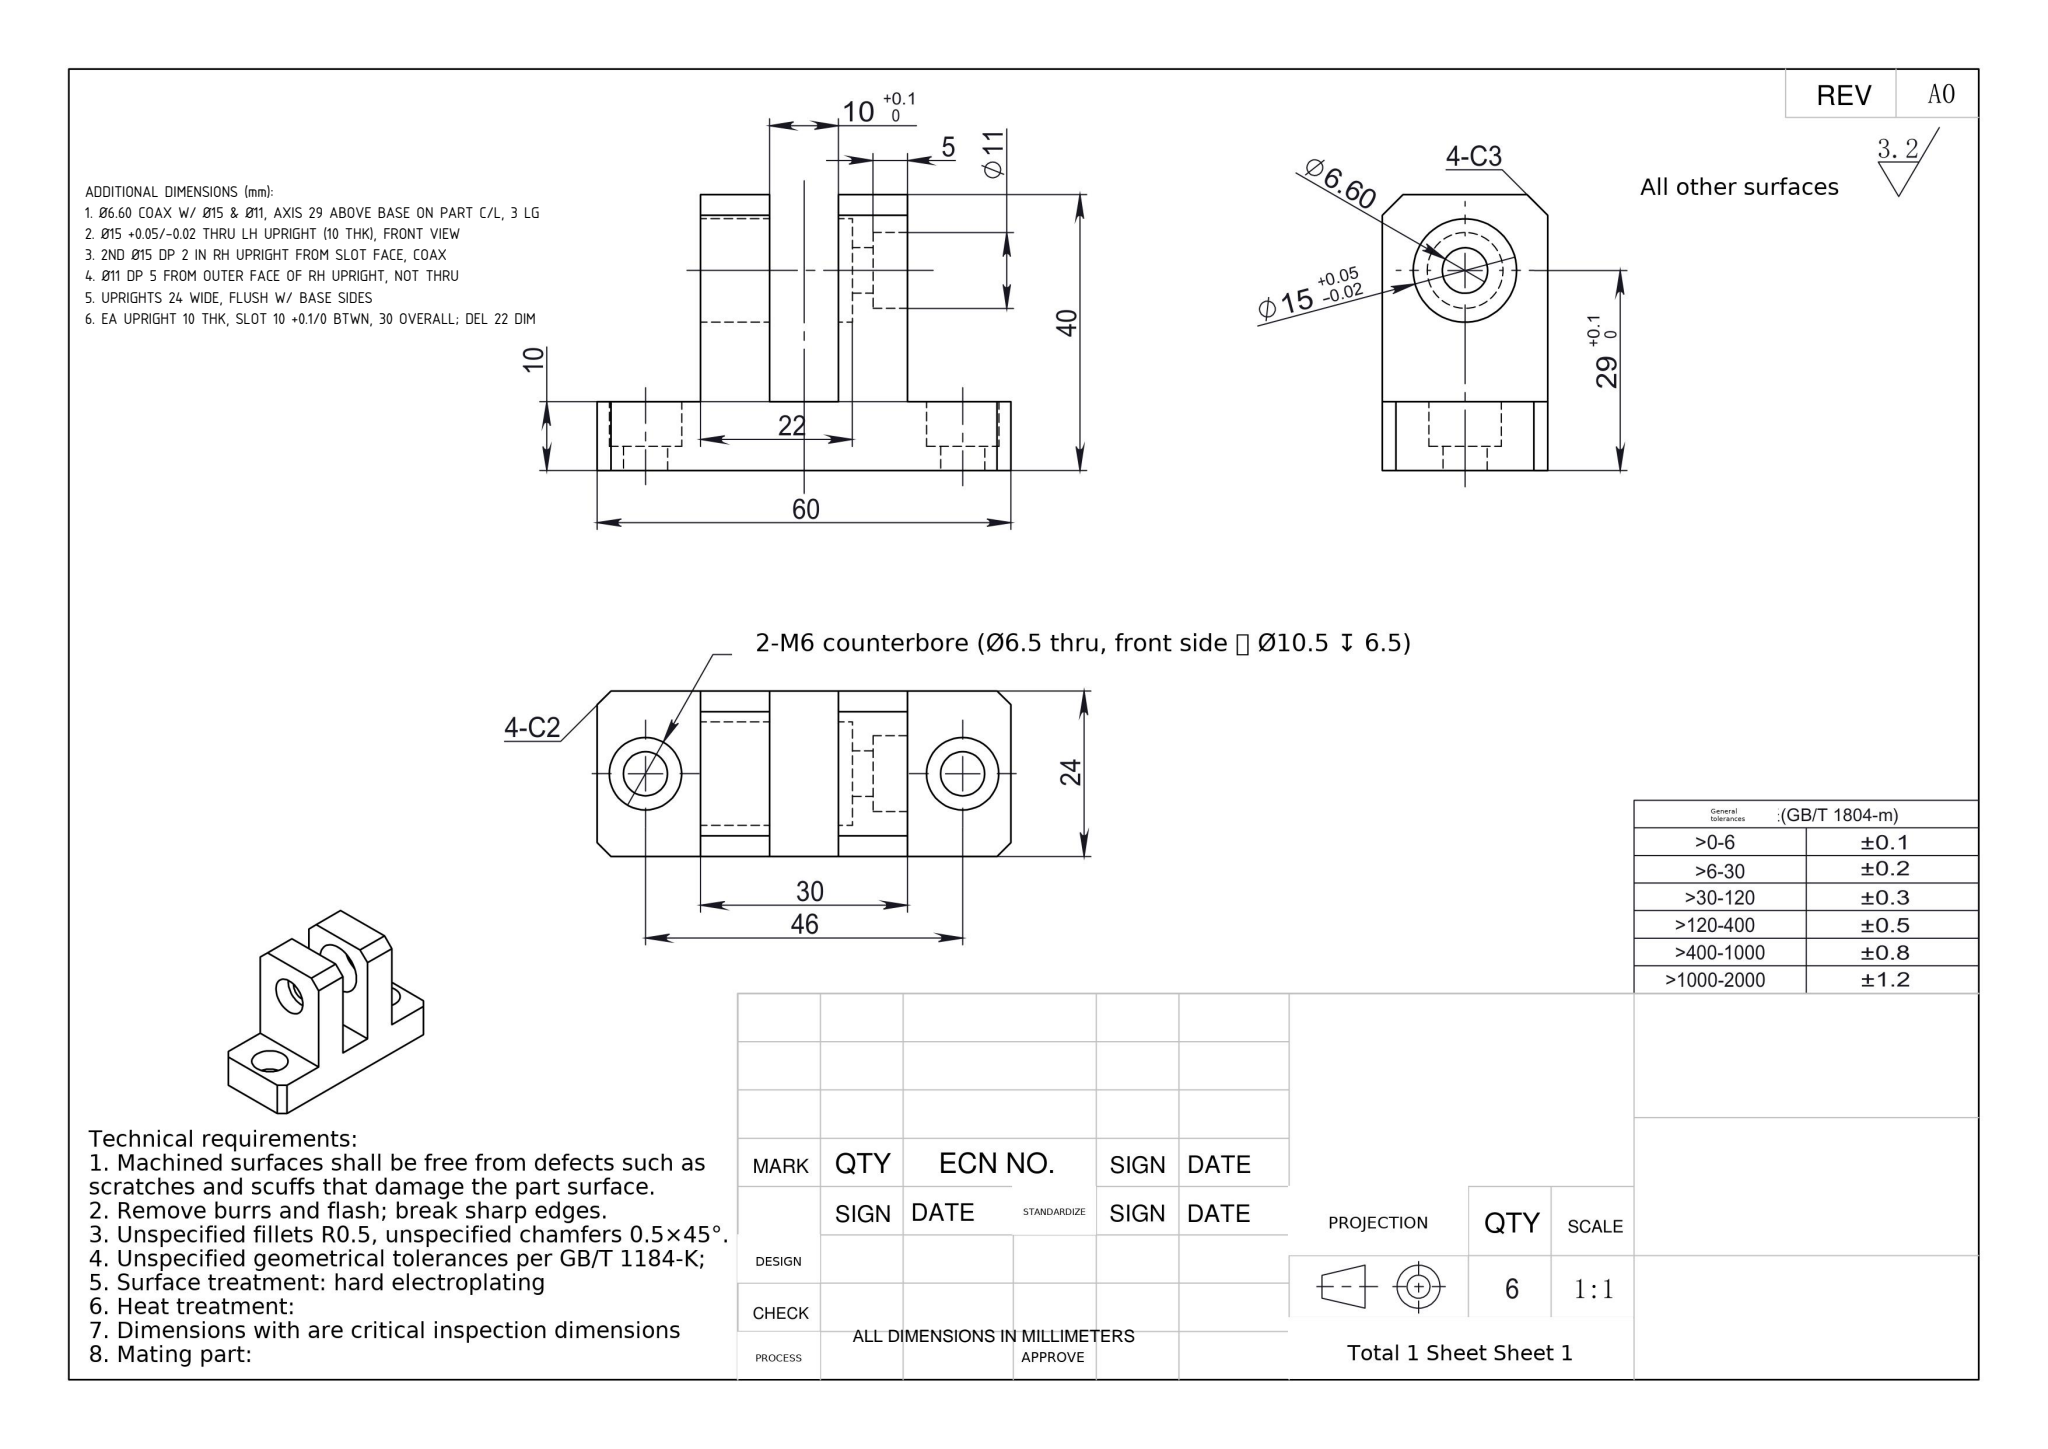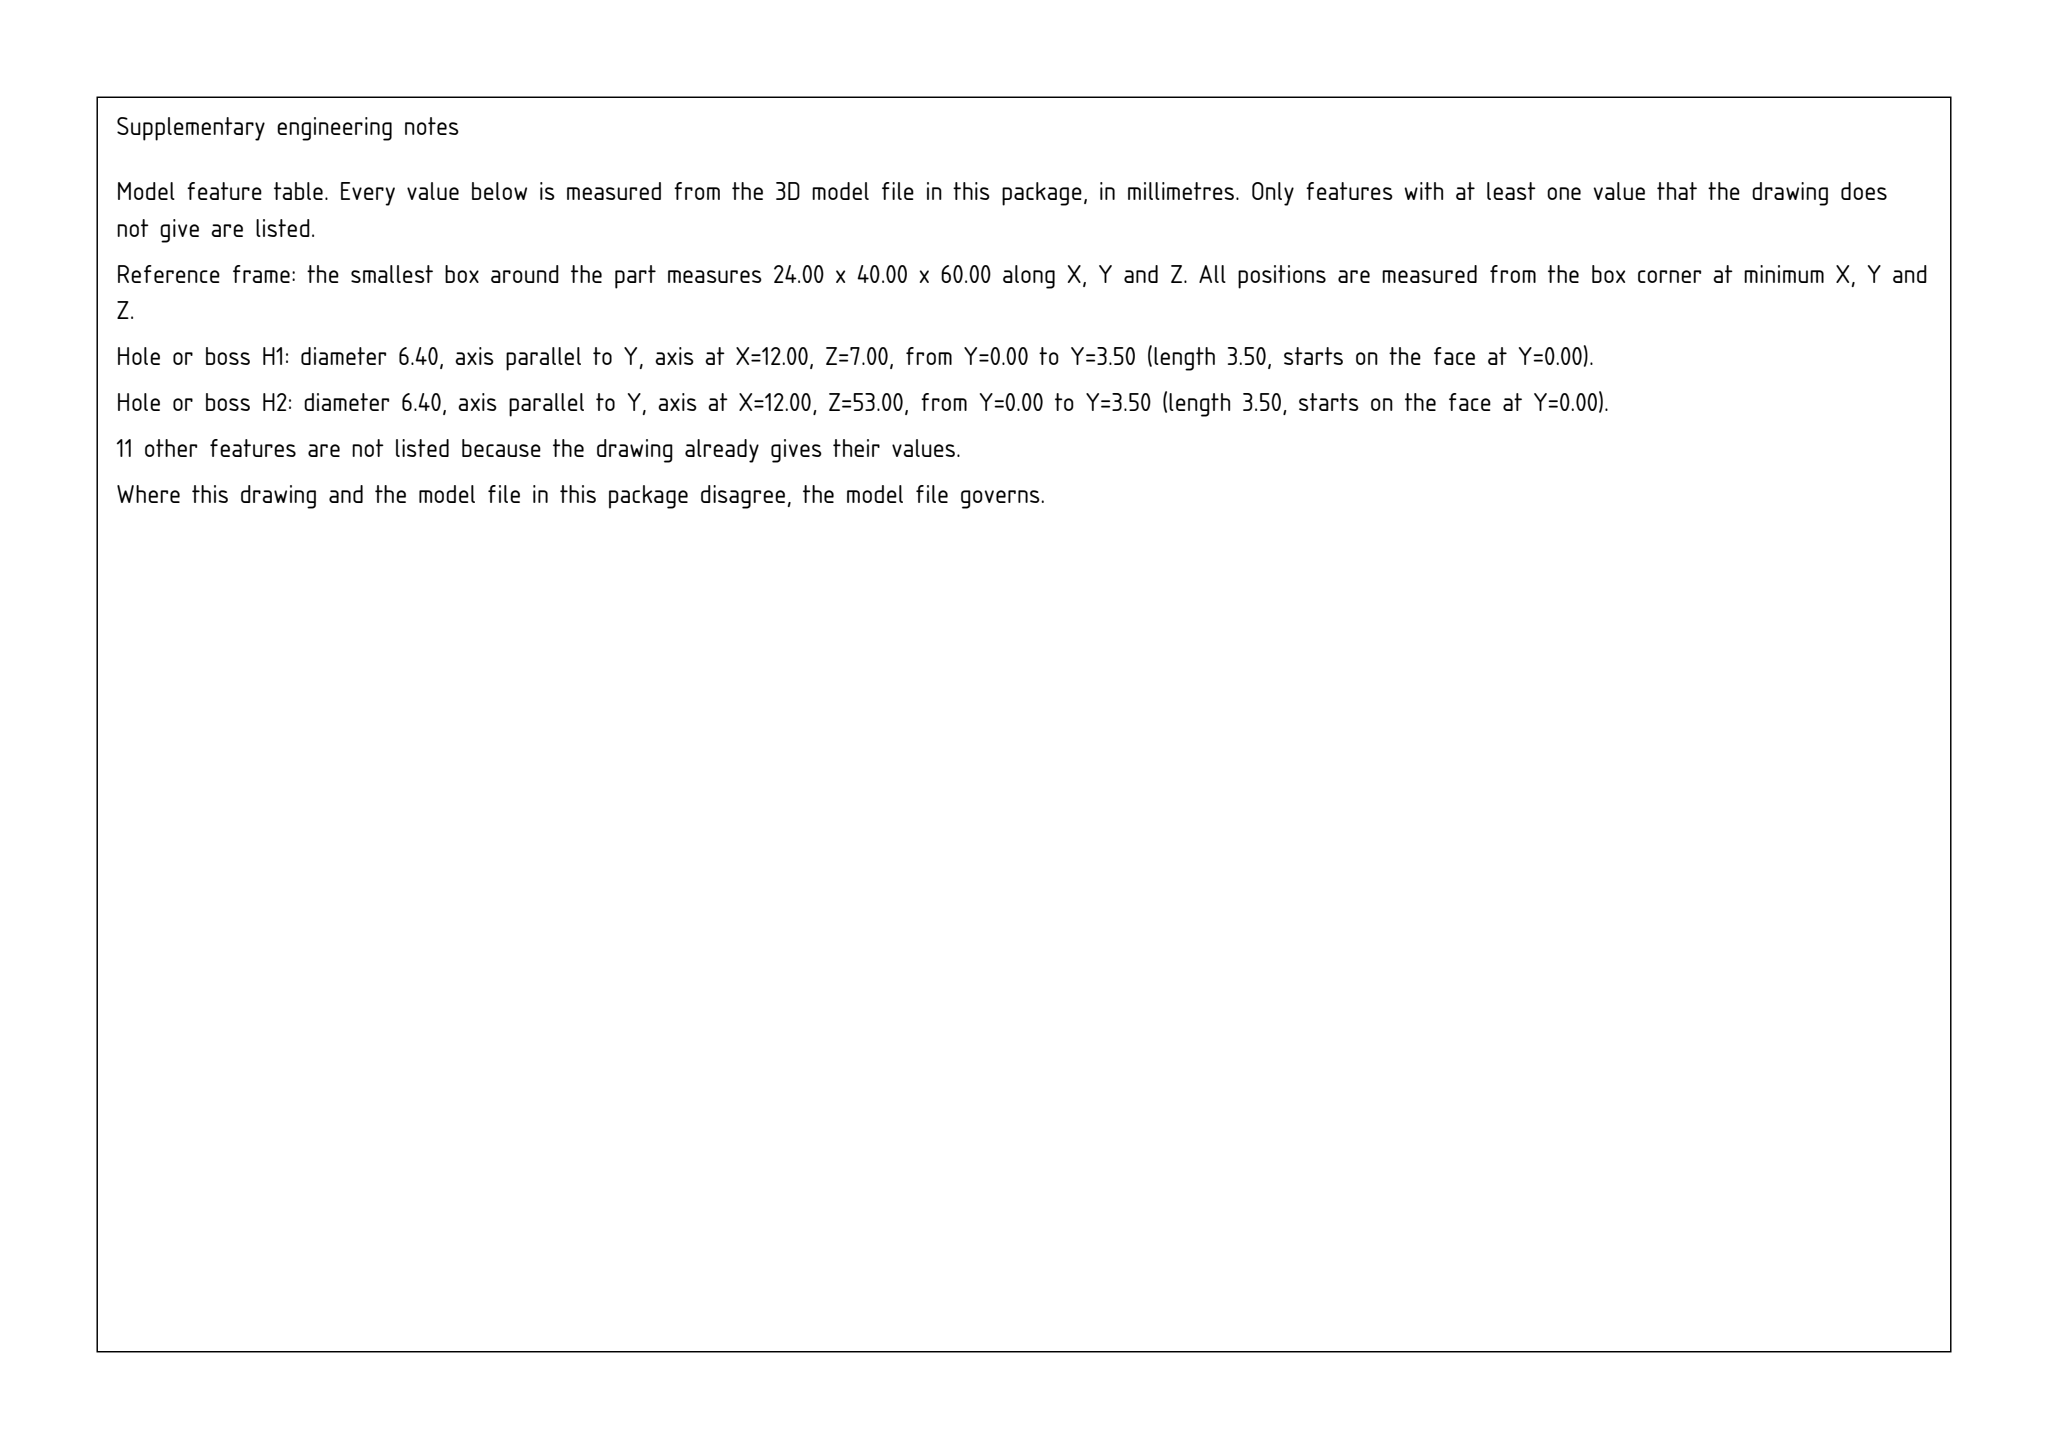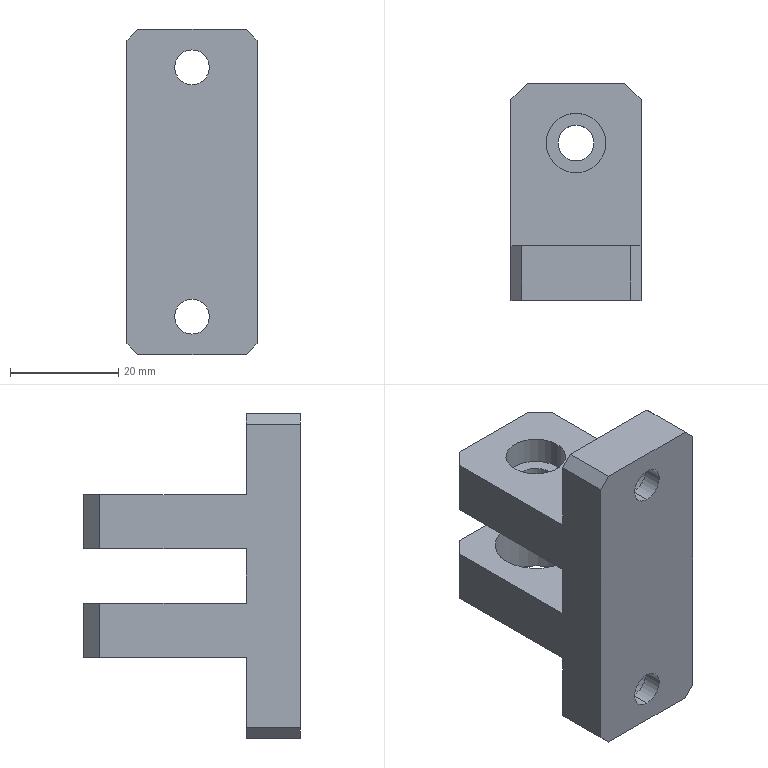Part | SolidWorks | mm | 1 solid | 42 faces | box 24 x 40 x 60 mm | volume 24491 mm3 | plane 26 | cylinder 16 | commonest cylinder face diameters 10.5 x4 6.4 x4 15 x4 11 x2 6.6 x2
build123d program:
from build123d import *

# Parameters (mm, degrees)
SKETCH1_W                                            = 24
SKETCH1_H                                            = 40
EXTRUDE1_DEPTH                                       = 30
SKETCH4_R                                            = 7.5
EXTRUDE4_DEPTH                                       = 22
CBORE_FOR_M6_HEXAGON_SOCKET_HEAD_CAP_SCR_D           = 6.6
CBORE_FOR_M6_HEXAGON_SOCKET_HEAD_CAP_SCR_DEPTH       = 25
CBORE_FOR_M6_HEXAGON_SOCKET_HEAD_CAP_SCR_CBORE_D     = 11
CBORE_FOR_M6_HEXAGON_SOCKET_HEAD_CAP_SCR_CBORE_DEPTH = 5
CBORE_FOR_M6_HEXAGON_SOCKET_HEAD_CAP_SCR_TIP         = 1.983
SKETCH7_W                                            = 10
SKETCH7_H                                            = 30
EXTRUDE5_DEPTH                                       = 44.313
SKETCH8_W                                            = 24
SKETCH8_H                                            = 60
EXTRUDE6_DEPTH                                       = 10
CBORE_FOR_M6_HEXAGON_SOCKET_HEAD_CAP_2_D             = 6.4
CBORE_FOR_M6_HEXAGON_SOCKET_HEAD_CAP_2_DEPTH         = 25
CBORE_FOR_M6_HEXAGON_SOCKET_HEAD_CAP_2_CBORE_D       = 10.5
CBORE_FOR_M6_HEXAGON_SOCKET_HEAD_CAP_2_CBORE_DEPTH   = 6.5
CBORE_FOR_M6_HEXAGON_SOCKET_HEAD_CAP_2_TIP           = 1.923
CHAMFER1_SIZE                                        = 2
CHAMFER2_SIZE                                        = 3


with BuildPart() as part:
    # Sketch1 → Extrude1 (new body)
    with BuildSketch(Plane.XY):
        Rectangle(SKETCH1_W, SKETCH1_H)
    extrude(amount=EXTRUDE1_DEPTH)

    # Sketch4 → Extrude4 (cut)
    with BuildSketch(Plane(origin=(0, 0, 0), x_dir=(-1, 0, 0), z_dir=(0, 0, -1))):
        with Locations((0, 9)):
            Circle(SKETCH4_R)
    extrude(amount=-EXTRUDE4_DEPTH, mode=Mode.SUBTRACT)

    # CBORE for M6 Hexagon socket head cap scr
    with Locations(Plane.XY.offset(30)):
        with Locations((0, 9)):
            CounterBoreHole(CBORE_FOR_M6_HEXAGON_SOCKET_HEAD_CAP_SCR_D / 2, CBORE_FOR_M6_HEXAGON_SOCKET_HEAD_CAP_SCR_CBORE_D / 2, CBORE_FOR_M6_HEXAGON_SOCKET_HEAD_CAP_SCR_CBORE_DEPTH, depth=CBORE_FOR_M6_HEXAGON_SOCKET_HEAD_CAP_SCR_DEPTH)
            with Locations((0, 0, -(CBORE_FOR_M6_HEXAGON_SOCKET_HEAD_CAP_SCR_DEPTH + CBORE_FOR_M6_HEXAGON_SOCKET_HEAD_CAP_SCR_TIP / 2))):  # 118° drill point
                Cone(0, CBORE_FOR_M6_HEXAGON_SOCKET_HEAD_CAP_SCR_D / 2, CBORE_FOR_M6_HEXAGON_SOCKET_HEAD_CAP_SCR_TIP, mode=Mode.SUBTRACT)

    # Sketch7 → Extrude5 (cut, through all)
    with BuildSketch(Plane.ZY.offset(12)):
        with Locations((15, 5)):
            Rectangle(SKETCH7_W, SKETCH7_H)
    extrude(amount=-EXTRUDE5_DEPTH, mode=Mode.SUBTRACT)

    # Sketch8 → Extrude6 (add)
    with BuildSketch(Plane.XZ.offset(20)):
        with Locations((0, 15)):
            Rectangle(SKETCH8_W, SKETCH8_H)
    extrude(amount=-EXTRUDE6_DEPTH)

    # CBORE for M6 Hexagon socket head cap 2
    with Locations(Plane(origin=(0, -10, 0), x_dir=(1, 0, 0), z_dir=(0, 1, 0))):
        with Locations((0, 8), (0, -38)):
            CounterBoreHole(CBORE_FOR_M6_HEXAGON_SOCKET_HEAD_CAP_2_D / 2, CBORE_FOR_M6_HEXAGON_SOCKET_HEAD_CAP_2_CBORE_D / 2, CBORE_FOR_M6_HEXAGON_SOCKET_HEAD_CAP_2_CBORE_DEPTH, depth=CBORE_FOR_M6_HEXAGON_SOCKET_HEAD_CAP_2_DEPTH)
            with Locations((0, 0, -(CBORE_FOR_M6_HEXAGON_SOCKET_HEAD_CAP_2_DEPTH + CBORE_FOR_M6_HEXAGON_SOCKET_HEAD_CAP_2_TIP / 2))):  # 118° drill point
                Cone(0, CBORE_FOR_M6_HEXAGON_SOCKET_HEAD_CAP_2_D / 2, CBORE_FOR_M6_HEXAGON_SOCKET_HEAD_CAP_2_TIP, mode=Mode.SUBTRACT)

    # Chamfer1
    chamfer1_edges = [part.edges().sort_by_distance(p)[0] for p in [
        (12, -15, 45),
        (-12, -15, -15),
        (-12, -15, 45),
        (12, -15, -15),
    ]]
    chamfer(chamfer1_edges, length=CHAMFER1_SIZE)

    # Chamfer2
    chamfer2_edges = [part.edges().sort_by_distance(p)[0] for p in [
        (-12, 20, 5),
        (12, 20, 5),
        (-12, 20, 25),
        (12, 20, 25),
    ]]
    chamfer(chamfer2_edges, length=CHAMFER2_SIZE)


solid = part.part